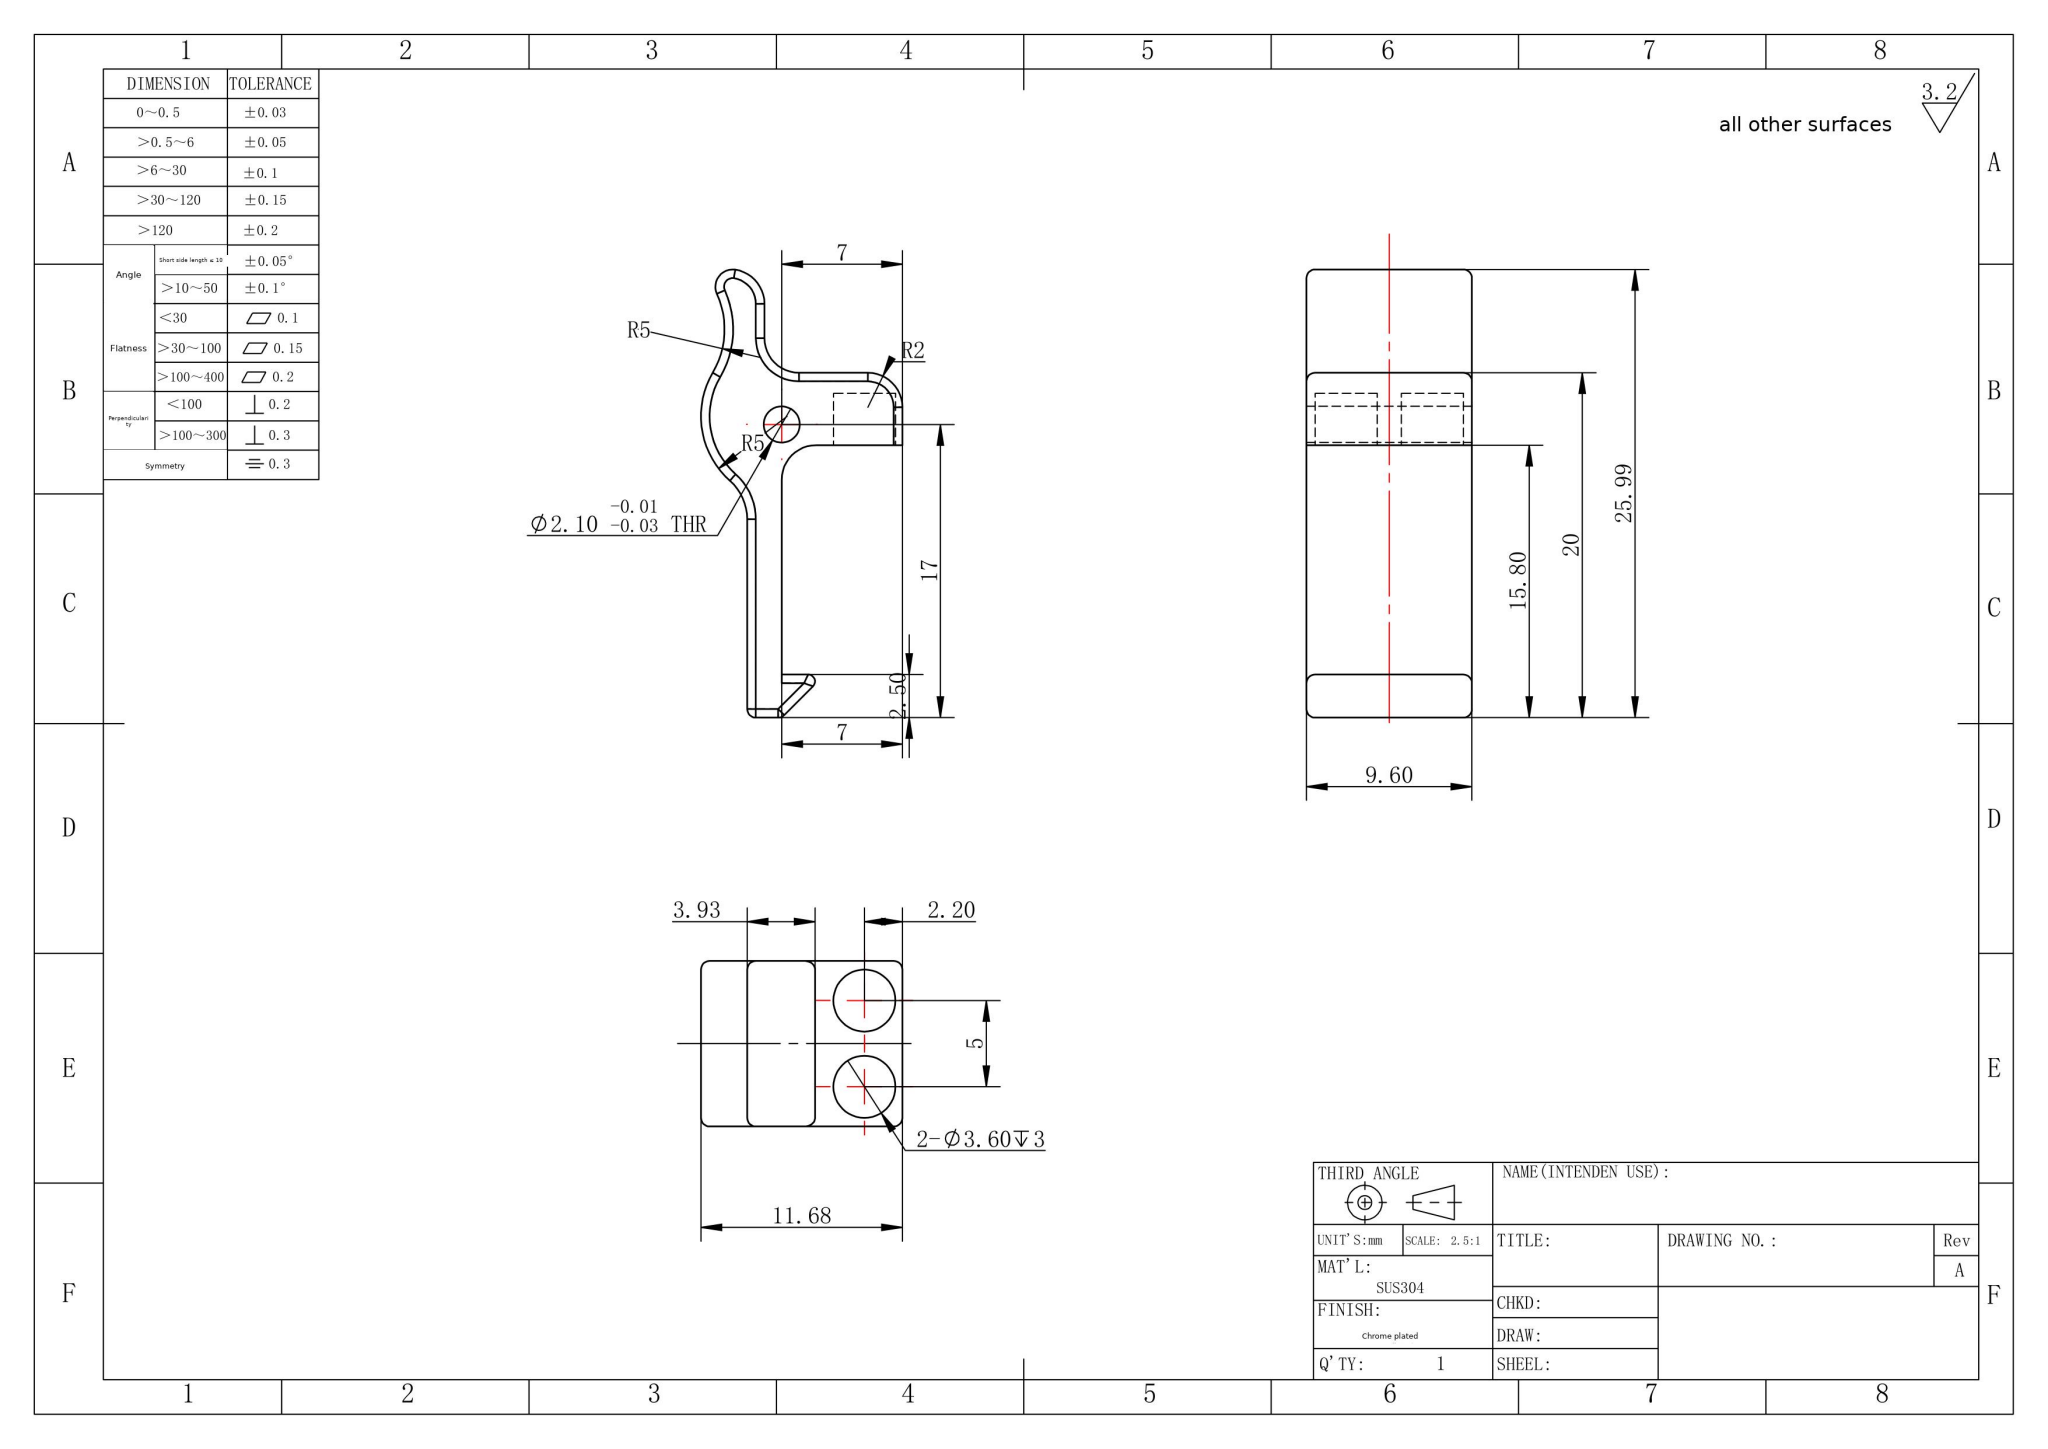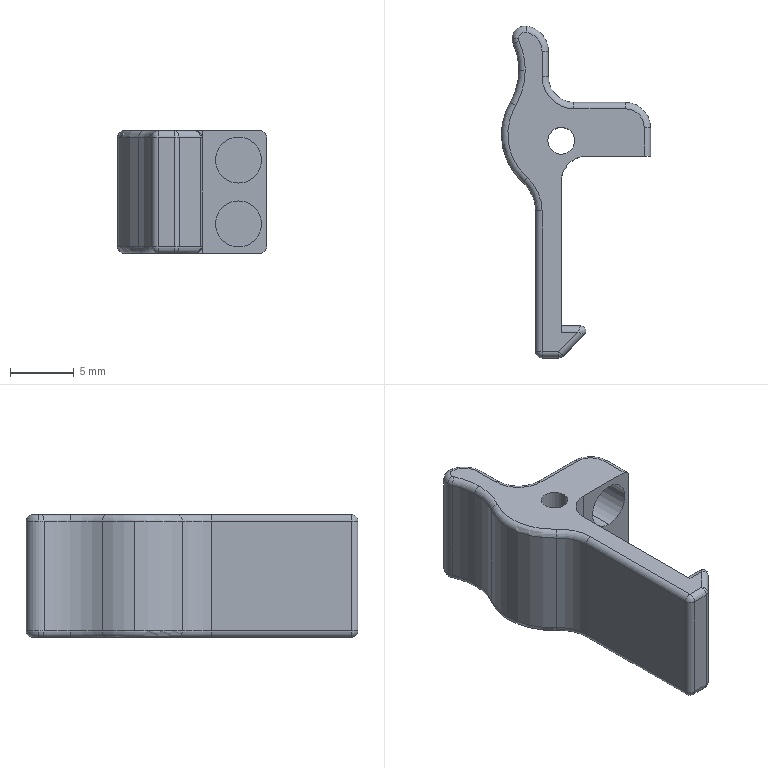Part | SolidWorks | mm | material SUS304 | 1 solid | 69 faces | box 11.68 x 25.99 x 9.6 mm | volume 885 mm3 | cylinder 32 | torus 18 | plane 13 | sphere 4 | spline 2 | commonest cylinder face diameters 1 x16 3.6 x4 4 x4 10 x3 2.1 x2 6 x1 2 x1 0.8 x1